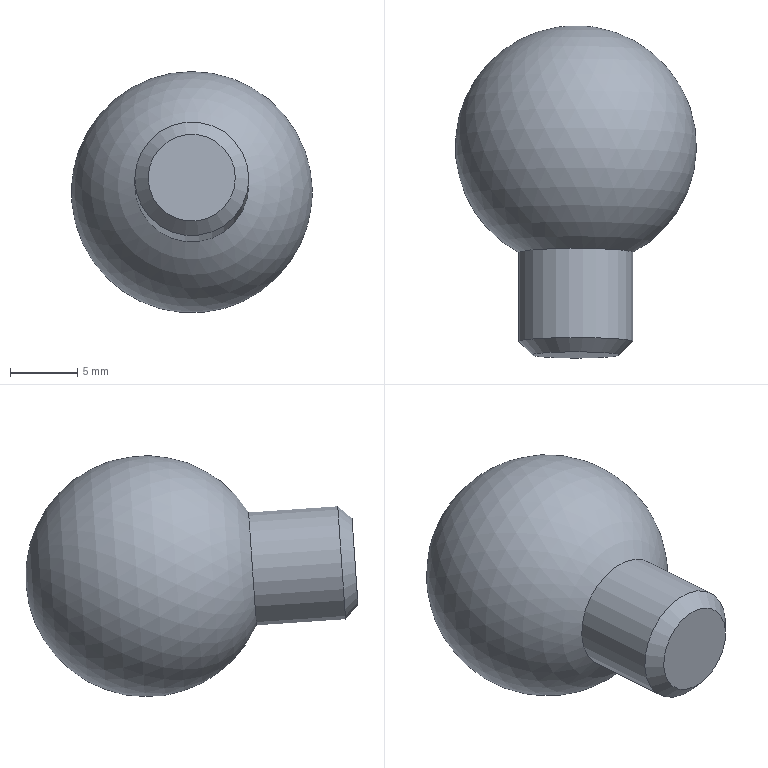Component | NX | PLUG | 1 solid | 4 faces | box 18 x 24.79 x 18 mm | volume 3445 mm3 | cylinder 1 | plane 1 | cone 1 | sphere 1 | commonest cylinder face diameters 8.5 x1
STEP:
#1=CARTESIAN_POINT('',(0.,0.,0.));
#2=DIRECTION('',(0.,0.,1.));
#3=DIRECTION('',(1.,0.,0.));
#4=AXIS2_PLACEMENT_3D('',#1,#2,#3);
#5=CARTESIAN_POINT('',(-18.441,56.095,-51.069));
#6=VERTEX_POINT('',#5);
#7=CARTESIAN_POINT('',(-9.941,56.095,-51.069));
#8=VERTEX_POINT('',#7);
#9=CARTESIAN_POINT('',(-14.191,56.095,-51.069));
#10=DIRECTION('',(0.,-0.9976,0.06885));
#11=DIRECTION('',(-1.,0.,0.));
#12=AXIS2_PLACEMENT_3D('',#9,#10,#11);
#13=CIRCLE('',#12,4.25);
#14=CARTESIAN_POINT('',(-14.191,48.447,-50.541));
#15=DIRECTION('',(0.,0.9976,-0.06885));
#16=DIRECTION('',(-1.,0.,0.));
#17=AXIS2_PLACEMENT_3D('',#14,#15,#16);
#18=CYLINDRICAL_SURFACE('',#17,4.25);
#19=CARTESIAN_POINT('',(6.283,7.667));
#20=DIRECTION('',(-1.,0.));
#21=VECTOR('',#20,1.);
#22=LINE('',#19,#21);
#23=(GEOMETRIC_REPRESENTATION_CONTEXT(2)PARAMETRIC_REPRESENTATION_CONTEXT()REPRESENTATION_CONTEXT('',''));
#24=DEFINITIONAL_REPRESENTATION('',(#22),#23);
#25=PCURVE('',#18,#24);
#26=CARTESIAN_POINT('',(-14.191,64.01,-51.615));
#27=DIRECTION('',(0.,-0.9976,0.06885));
#28=DIRECTION('',(1.,0.,0.));
#29=AXIS2_PLACEMENT_3D('',#26,#27,#28);
#30=SPHERICAL_SURFACE('',#29,9.);
#31=CARTESIAN_POINT('',(3.142,1.079));
#32=CARTESIAN_POINT('',(3.237,1.079));
#33=CARTESIAN_POINT('',(3.427,1.079));
#34=CARTESIAN_POINT('',(3.713,1.079));
#35=CARTESIAN_POINT('',(3.998,1.079));
#36=CARTESIAN_POINT('',(4.284,1.079));
#37=CARTESIAN_POINT('',(4.57,1.079));
#38=CARTESIAN_POINT('',(4.855,1.079));
#39=CARTESIAN_POINT('',(5.141,1.079));
#40=CARTESIAN_POINT('',(5.426,1.079));
#41=CARTESIAN_POINT('',(5.712,1.079));
#42=CARTESIAN_POINT('',(5.998,1.079));
#43=CARTESIAN_POINT('',(6.283,1.079));
#44=CARTESIAN_POINT('',(6.569,1.079));
#45=CARTESIAN_POINT('',(6.854,1.079));
#46=CARTESIAN_POINT('',(7.14,1.079));
#47=CARTESIAN_POINT('',(7.426,1.079));
#48=CARTESIAN_POINT('',(7.711,1.079));
#49=CARTESIAN_POINT('',(7.997,1.079));
#50=CARTESIAN_POINT('',(8.282,1.079));
#51=CARTESIAN_POINT('',(8.568,1.079));
#52=CARTESIAN_POINT('',(8.854,1.079));
#53=CARTESIAN_POINT('',(9.139,1.079));
#54=CARTESIAN_POINT('',(9.33,1.079));
#55=CARTESIAN_POINT('',(9.425,1.079));
#56=B_SPLINE_CURVE_WITH_KNOTS('',3,(#31,#32,#33,#34,#35,#36,#37,#38,#39,#40,#41,#42,#43,#44,#45,#46,#47,#48,#49,#50,#51,#52,#53,#54,#55),.UNSPECIFIED.,.F.,.F.,(4,1,1,1,1,1,1,1,1,1,1,1,1,1,1,1,1,1,1,1,1,1,4),(0.,0.2856,0.5712,0.8568,1.142,1.428,1.714,1.999,2.285,2.57,2.856,3.142,3.427,3.713,3.998,4.284,4.57,4.855,5.141,5.426,5.712,5.998,6.283),.QUASI_UNIFORM_KNOTS.);
#57=(GEOMETRIC_REPRESENTATION_CONTEXT(2)PARAMETRIC_REPRESENTATION_CONTEXT()REPRESENTATION_CONTEXT('',''));
#58=DEFINITIONAL_REPRESENTATION('',(#56),#57);
#59=PCURVE('',#30,#58);
#60=SURFACE_CURVE('',#13,(#25,#59),.PCURVE_S1.);
#61=EDGE_CURVE('',#6,#8,#60,.T.);
#62=ORIENTED_EDGE('',*,*,#61,.T.);
#63=CARTESIAN_POINT('',(-14.191,56.095,-51.069));
#64=DIRECTION('',(0.,-0.9976,0.06885));
#65=DIRECTION('',(-1.,0.,0.));
#66=AXIS2_PLACEMENT_3D('',#63,#64,#65);
#67=CIRCLE('',#66,4.25);
#68=CARTESIAN_POINT('',(6.283,7.667));
#69=DIRECTION('',(-1.,0.));
#70=VECTOR('',#69,1.);
#71=LINE('',#68,#70);
#72=(GEOMETRIC_REPRESENTATION_CONTEXT(2)PARAMETRIC_REPRESENTATION_CONTEXT()REPRESENTATION_CONTEXT('',''));
#73=DEFINITIONAL_REPRESENTATION('',(#71),#72);
#74=PCURVE('',#18,#73);
#75=CARTESIAN_POINT('',(-3.142,1.079));
#76=CARTESIAN_POINT('',(-3.046,1.079));
#77=CARTESIAN_POINT('',(-2.856,1.079));
#78=CARTESIAN_POINT('',(-2.57,1.079));
#79=CARTESIAN_POINT('',(-2.285,1.079));
#80=CARTESIAN_POINT('',(-1.999,1.079));
#81=CARTESIAN_POINT('',(-1.714,1.079));
#82=CARTESIAN_POINT('',(-1.428,1.079));
#83=CARTESIAN_POINT('',(-1.142,1.079));
#84=CARTESIAN_POINT('',(-0.8568,1.079));
#85=CARTESIAN_POINT('',(-0.5712,1.079));
#86=CARTESIAN_POINT('',(-0.2856,1.079));
#87=CARTESIAN_POINT('',(0.,1.079));
#88=CARTESIAN_POINT('',(0.2856,1.079));
#89=CARTESIAN_POINT('',(0.5712,1.079));
#90=CARTESIAN_POINT('',(0.8568,1.079));
#91=CARTESIAN_POINT('',(1.142,1.079));
#92=CARTESIAN_POINT('',(1.428,1.079));
#93=CARTESIAN_POINT('',(1.714,1.079));
#94=CARTESIAN_POINT('',(1.999,1.079));
#95=CARTESIAN_POINT('',(2.285,1.079));
#96=CARTESIAN_POINT('',(2.57,1.079));
#97=CARTESIAN_POINT('',(2.856,1.079));
#98=CARTESIAN_POINT('',(3.046,1.079));
#99=CARTESIAN_POINT('',(3.142,1.079));
#100=B_SPLINE_CURVE_WITH_KNOTS('',3,(#75,#76,#77,#78,#79,#80,#81,#82,#83,#84,#85,#86,#87,#88,#89,#90,#91,#92,#93,#94,#95,#96,#97,#98,#99),.UNSPECIFIED.,.F.,.F.,(4,1,1,1,1,1,1,1,1,1,1,1,1,1,1,1,1,1,1,1,1,1,4),(0.,0.2856,0.5712,0.8568,1.142,1.428,1.714,1.999,2.285,2.57,2.856,3.142,3.427,3.713,3.998,4.284,4.57,4.855,5.141,5.426,5.712,5.998,6.283),.QUASI_UNIFORM_KNOTS.);
#101=(GEOMETRIC_REPRESENTATION_CONTEXT(2)PARAMETRIC_REPRESENTATION_CONTEXT()REPRESENTATION_CONTEXT('',''));
#102=DEFINITIONAL_REPRESENTATION('',(#100),#101);
#103=PCURVE('',#30,#102);
#104=SURFACE_CURVE('',#67,(#74,#103),.PCURVE_S1.);
#105=EDGE_CURVE('',#8,#6,#104,.T.);
#106=ORIENTED_EDGE('',*,*,#105,.T.);
#107=CARTESIAN_POINT('',(-18.441,49.445,-50.61));
#108=VERTEX_POINT('',#107);
#109=CARTESIAN_POINT('',(-18.441,49.445,-50.61));
#110=CARTESIAN_POINT('',(-18.441,56.095,-51.069));
#111=B_SPLINE_CURVE_WITH_KNOTS('',1,(#109,#110),.UNSPECIFIED.,.F.,.F.,(2,2),(1.,7.667),.PIECEWISE_BEZIER_KNOTS.);
#112=CARTESIAN_POINT('',(0.,0.));
#113=DIRECTION('',(0.,1.));
#114=VECTOR('',#113,1.);
#115=LINE('',#112,#114);
#116=(GEOMETRIC_REPRESENTATION_CONTEXT(2)PARAMETRIC_REPRESENTATION_CONTEXT()REPRESENTATION_CONTEXT('',''));
#117=DEFINITIONAL_REPRESENTATION('',(#115),#116);
#118=PCURVE('',#18,#117);
#119=CARTESIAN_POINT('',(6.283,0.));
#120=DIRECTION('',(0.,1.));
#121=VECTOR('',#120,1.);
#122=LINE('',#119,#121);
#123=(GEOMETRIC_REPRESENTATION_CONTEXT(2)PARAMETRIC_REPRESENTATION_CONTEXT()REPRESENTATION_CONTEXT('',''));
#124=DEFINITIONAL_REPRESENTATION('',(#122),#123);
#125=PCURVE('',#18,#124);
#126=SEAM_CURVE('',#111,(#118,#125),.PCURVE_S1.);
#127=EDGE_CURVE('',#108,#6,#126,.T.);
#128=ORIENTED_EDGE('',*,*,#127,.F.);
#129=CARTESIAN_POINT('',(-9.941,49.445,-50.61));
#130=VERTEX_POINT('',#129);
#131=CARTESIAN_POINT('',(-14.191,49.445,-50.61));
#132=DIRECTION('',(0.,0.9976,-0.06885));
#133=DIRECTION('',(1.,0.,0.));
#134=AXIS2_PLACEMENT_3D('',#131,#132,#133);
#135=CIRCLE('',#134,4.25);
#136=CARTESIAN_POINT('',(-3.142,1.));
#137=DIRECTION('',(1.,0.));
#138=VECTOR('',#137,1.);
#139=LINE('',#136,#138);
#140=(GEOMETRIC_REPRESENTATION_CONTEXT(2)PARAMETRIC_REPRESENTATION_CONTEXT()REPRESENTATION_CONTEXT('',''));
#141=DEFINITIONAL_REPRESENTATION('',(#139),#140);
#142=PCURVE('',#18,#141);
#143=CARTESIAN_POINT('',(-14.191,48.447,-50.541));
#144=DIRECTION('',(0.,0.9976,-0.06885));
#145=DIRECTION('',(-1.,-0.,-0.));
#146=AXIS2_PLACEMENT_3D('',#143,#144,#145);
#147=CONICAL_SURFACE('',#146,3.25,0.7854);
#148=CARTESIAN_POINT('',(3.142,1.));
#149=DIRECTION('',(1.,-0.));
#150=VECTOR('',#149,1.);
#151=LINE('',#148,#150);
#152=(GEOMETRIC_REPRESENTATION_CONTEXT(2)PARAMETRIC_REPRESENTATION_CONTEXT()REPRESENTATION_CONTEXT('',''));
#153=DEFINITIONAL_REPRESENTATION('',(#151),#152);
#154=PCURVE('',#147,#153);
#155=SURFACE_CURVE('',#135,(#142,#154),.PCURVE_S1.);
#156=EDGE_CURVE('',#108,#130,#155,.T.);
#157=ORIENTED_EDGE('',*,*,#156,.T.);
#158=CARTESIAN_POINT('',(-14.191,49.445,-50.61));
#159=DIRECTION('',(0.,0.9976,-0.06885));
#160=DIRECTION('',(1.,0.,0.));
#161=AXIS2_PLACEMENT_3D('',#158,#159,#160);
#162=CIRCLE('',#161,4.25);
#163=CARTESIAN_POINT('',(3.142,1.));
#164=DIRECTION('',(1.,0.));
#165=VECTOR('',#164,1.);
#166=LINE('',#163,#165);
#167=(GEOMETRIC_REPRESENTATION_CONTEXT(2)PARAMETRIC_REPRESENTATION_CONTEXT()REPRESENTATION_CONTEXT('',''));
#168=DEFINITIONAL_REPRESENTATION('',(#166),#167);
#169=PCURVE('',#18,#168);
#170=CARTESIAN_POINT('',(3.142,1.));
#171=DIRECTION('',(1.,0.));
#172=VECTOR('',#171,1.);
#173=LINE('',#170,#172);
#174=(GEOMETRIC_REPRESENTATION_CONTEXT(2)PARAMETRIC_REPRESENTATION_CONTEXT()REPRESENTATION_CONTEXT('',''));
#175=DEFINITIONAL_REPRESENTATION('',(#173),#174);
#176=PCURVE('',#147,#175);
#177=SURFACE_CURVE('',#162,(#169,#176),.PCURVE_S1.);
#178=EDGE_CURVE('',#130,#108,#177,.T.);
#179=ORIENTED_EDGE('',*,*,#178,.T.);
#180=ORIENTED_EDGE('',*,*,#127,.T.);
#181=EDGE_LOOP('',(#62,#106,#128,#157,#179,#180));
#182=FACE_BOUND('',#181,.T.);
#183=ADVANCED_FACE('',(#182),#18,.T.);
#184=CARTESIAN_POINT('',(-10.941,48.447,-50.541));
#185=VERTEX_POINT('',#184);
#186=CARTESIAN_POINT('',(-14.191,48.447,-50.541));
#187=DIRECTION('',(0.,-0.9976,0.06885));
#188=DIRECTION('',(1.,0.,0.));
#189=AXIS2_PLACEMENT_3D('',#186,#187,#188);
#190=CIRCLE('',#189,3.25);
#191=CARTESIAN_POINT('',(-14.191,48.447,-50.541));
#192=DIRECTION('',(0.,-0.9976,0.06885));
#193=DIRECTION('',(1.,0.,0.));
#194=AXIS2_PLACEMENT_3D('',#191,#192,#193);
#195=PLANE('',#194);
#196=CARTESIAN_POINT('',(0.,0.));
#197=DIRECTION('',(1.,0.));
#198=AXIS2_PLACEMENT_2D('',#196,#197);
#199=CIRCLE('',#198,3.25);
#200=(GEOMETRIC_REPRESENTATION_CONTEXT(2)PARAMETRIC_REPRESENTATION_CONTEXT()REPRESENTATION_CONTEXT('',''));
#201=DEFINITIONAL_REPRESENTATION('',(#199),#200);
#202=PCURVE('',#195,#201);
#203=CARTESIAN_POINT('',(9.425,0.));
#204=DIRECTION('',(-1.,0.));
#205=VECTOR('',#204,1.);
#206=LINE('',#203,#205);
#207=(GEOMETRIC_REPRESENTATION_CONTEXT(2)PARAMETRIC_REPRESENTATION_CONTEXT()REPRESENTATION_CONTEXT('',''));
#208=DEFINITIONAL_REPRESENTATION('',(#206),#207);
#209=PCURVE('',#147,#208);
#210=SURFACE_CURVE('',#190,(#202,#209),.PCURVE_S1.);
#211=EDGE_CURVE('',#185,#185,#210,.T.);
#212=ORIENTED_EDGE('',*,*,#211,.T.);
#213=EDGE_LOOP('',(#212));
#214=FACE_BOUND('',#213,.T.);
#215=ADVANCED_FACE('',(#214),#195,.T.);
#216=ORIENTED_EDGE('',*,*,#178,.F.);
#217=CARTESIAN_POINT('',(-10.941,48.447,-50.541));
#218=CARTESIAN_POINT('',(-9.941,49.445,-50.61));
#219=B_SPLINE_CURVE_WITH_KNOTS('',1,(#217,#218),.UNSPECIFIED.,.F.,.F.,(2,2),(0.,1.414),.PIECEWISE_BEZIER_KNOTS.);
#220=CARTESIAN_POINT('',(3.142,0.));
#221=DIRECTION('',(0.,1.));
#222=VECTOR('',#221,1.);
#223=LINE('',#220,#222);
#224=(GEOMETRIC_REPRESENTATION_CONTEXT(2)PARAMETRIC_REPRESENTATION_CONTEXT()REPRESENTATION_CONTEXT('',''));
#225=DEFINITIONAL_REPRESENTATION('',(#223),#224);
#226=PCURVE('',#147,#225);
#227=CARTESIAN_POINT('',(9.425,0.));
#228=DIRECTION('',(0.,1.));
#229=VECTOR('',#228,1.);
#230=LINE('',#227,#229);
#231=(GEOMETRIC_REPRESENTATION_CONTEXT(2)PARAMETRIC_REPRESENTATION_CONTEXT()REPRESENTATION_CONTEXT('',''));
#232=DEFINITIONAL_REPRESENTATION('',(#230),#231);
#233=PCURVE('',#147,#232);
#234=SEAM_CURVE('',#219,(#226,#233),.PCURVE_S1.);
#235=EDGE_CURVE('',#185,#130,#234,.T.);
#236=ORIENTED_EDGE('',*,*,#235,.F.);
#237=ORIENTED_EDGE('',*,*,#211,.F.);
#238=ORIENTED_EDGE('',*,*,#235,.T.);
#239=ORIENTED_EDGE('',*,*,#156,.F.);
#240=EDGE_LOOP('',(#216,#236,#237,#238,#239));
#241=FACE_BOUND('',#240,.T.);
#242=ADVANCED_FACE('',(#241),#147,.T.);
#243=ORIENTED_EDGE('',*,*,#105,.F.);
#244=CARTESIAN_POINT('',(-14.191,72.989,-52.235));
#245=VERTEX_POINT('',#244);
#246=CARTESIAN_POINT('',(-14.191,72.989,-52.235));
#247=CARTESIAN_POINT('',(-11.21,72.989,-52.235));
#248=CARTESIAN_POINT('',(-8.229,71.863,-52.157));
#249=CARTESIAN_POINT('',(-5.747,69.612,-52.002));
#250=CARTESIAN_POINT('',(-4.26,66.497,-51.787));
#251=CARTESIAN_POINT('',(-4.096,63.05,-51.549));
#252=CARTESIAN_POINT('',(-5.219,59.897,-51.331));
#253=CARTESIAN_POINT('',(-7.314,57.5,-51.166));
#254=CARTESIAN_POINT('',(-9.941,56.095,-51.069));
#255=B_SPLINE_CURVE_WITH_KNOTS('',8,(#246,#247,#248,#249,#250,#251,#252,#253,#254),.UNSPECIFIED.,.F.,.F.,(9,9),(-1.571,1.079),.PIECEWISE_BEZIER_KNOTS.);
#256=CARTESIAN_POINT('',(0.,0.));
#257=DIRECTION('',(0.,1.));
#258=VECTOR('',#257,1.);
#259=LINE('',#256,#258);
#260=(GEOMETRIC_REPRESENTATION_CONTEXT(2)PARAMETRIC_REPRESENTATION_CONTEXT()REPRESENTATION_CONTEXT('',''));
#261=DEFINITIONAL_REPRESENTATION('',(#259),#260);
#262=PCURVE('',#30,#261);
#263=CARTESIAN_POINT('',(6.283,0.));
#264=DIRECTION('',(0.,1.));
#265=VECTOR('',#264,1.);
#266=LINE('',#263,#265);
#267=(GEOMETRIC_REPRESENTATION_CONTEXT(2)PARAMETRIC_REPRESENTATION_CONTEXT()REPRESENTATION_CONTEXT('',''));
#268=DEFINITIONAL_REPRESENTATION('',(#266),#267);
#269=PCURVE('',#30,#268);
#270=SEAM_CURVE('',#255,(#262,#269),.PCURVE_S1.);
#271=EDGE_CURVE('',#245,#8,#270,.T.);
#272=ORIENTED_EDGE('',*,*,#271,.F.);
#273=ORIENTED_EDGE('',*,*,#271,.T.);
#274=ORIENTED_EDGE('',*,*,#61,.F.);
#275=EDGE_LOOP('',(#243,#272,#273,#274));
#276=FACE_BOUND('',#275,.T.);
#277=ADVANCED_FACE('',(#276),#30,.T.);
#278=CLOSED_SHELL('',(#183,#215,#242,#277));
#279=MANIFOLD_SOLID_BREP('',#278);
#280=(LENGTH_UNIT()NAMED_UNIT(*)SI_UNIT(.MILLI.,.METRE.));
#281=UNCERTAINTY_MEASURE_WITH_UNIT(LENGTH_MEASURE(0.00001),#280,'','');
#282=(NAMED_UNIT(*)PLANE_ANGLE_UNIT()SI_UNIT($,.RADIAN.));
#283=(NAMED_UNIT(*)SI_UNIT($,.STERADIAN.)SOLID_ANGLE_UNIT());
#284=(GEOMETRIC_REPRESENTATION_CONTEXT(3)GLOBAL_UNCERTAINTY_ASSIGNED_CONTEXT((#281))GLOBAL_UNIT_ASSIGNED_CONTEXT((#280,#282,#283))REPRESENTATION_CONTEXT('',''));
#285=ADVANCED_BREP_SHAPE_REPRESENTATION('',(#4,#279),#284);